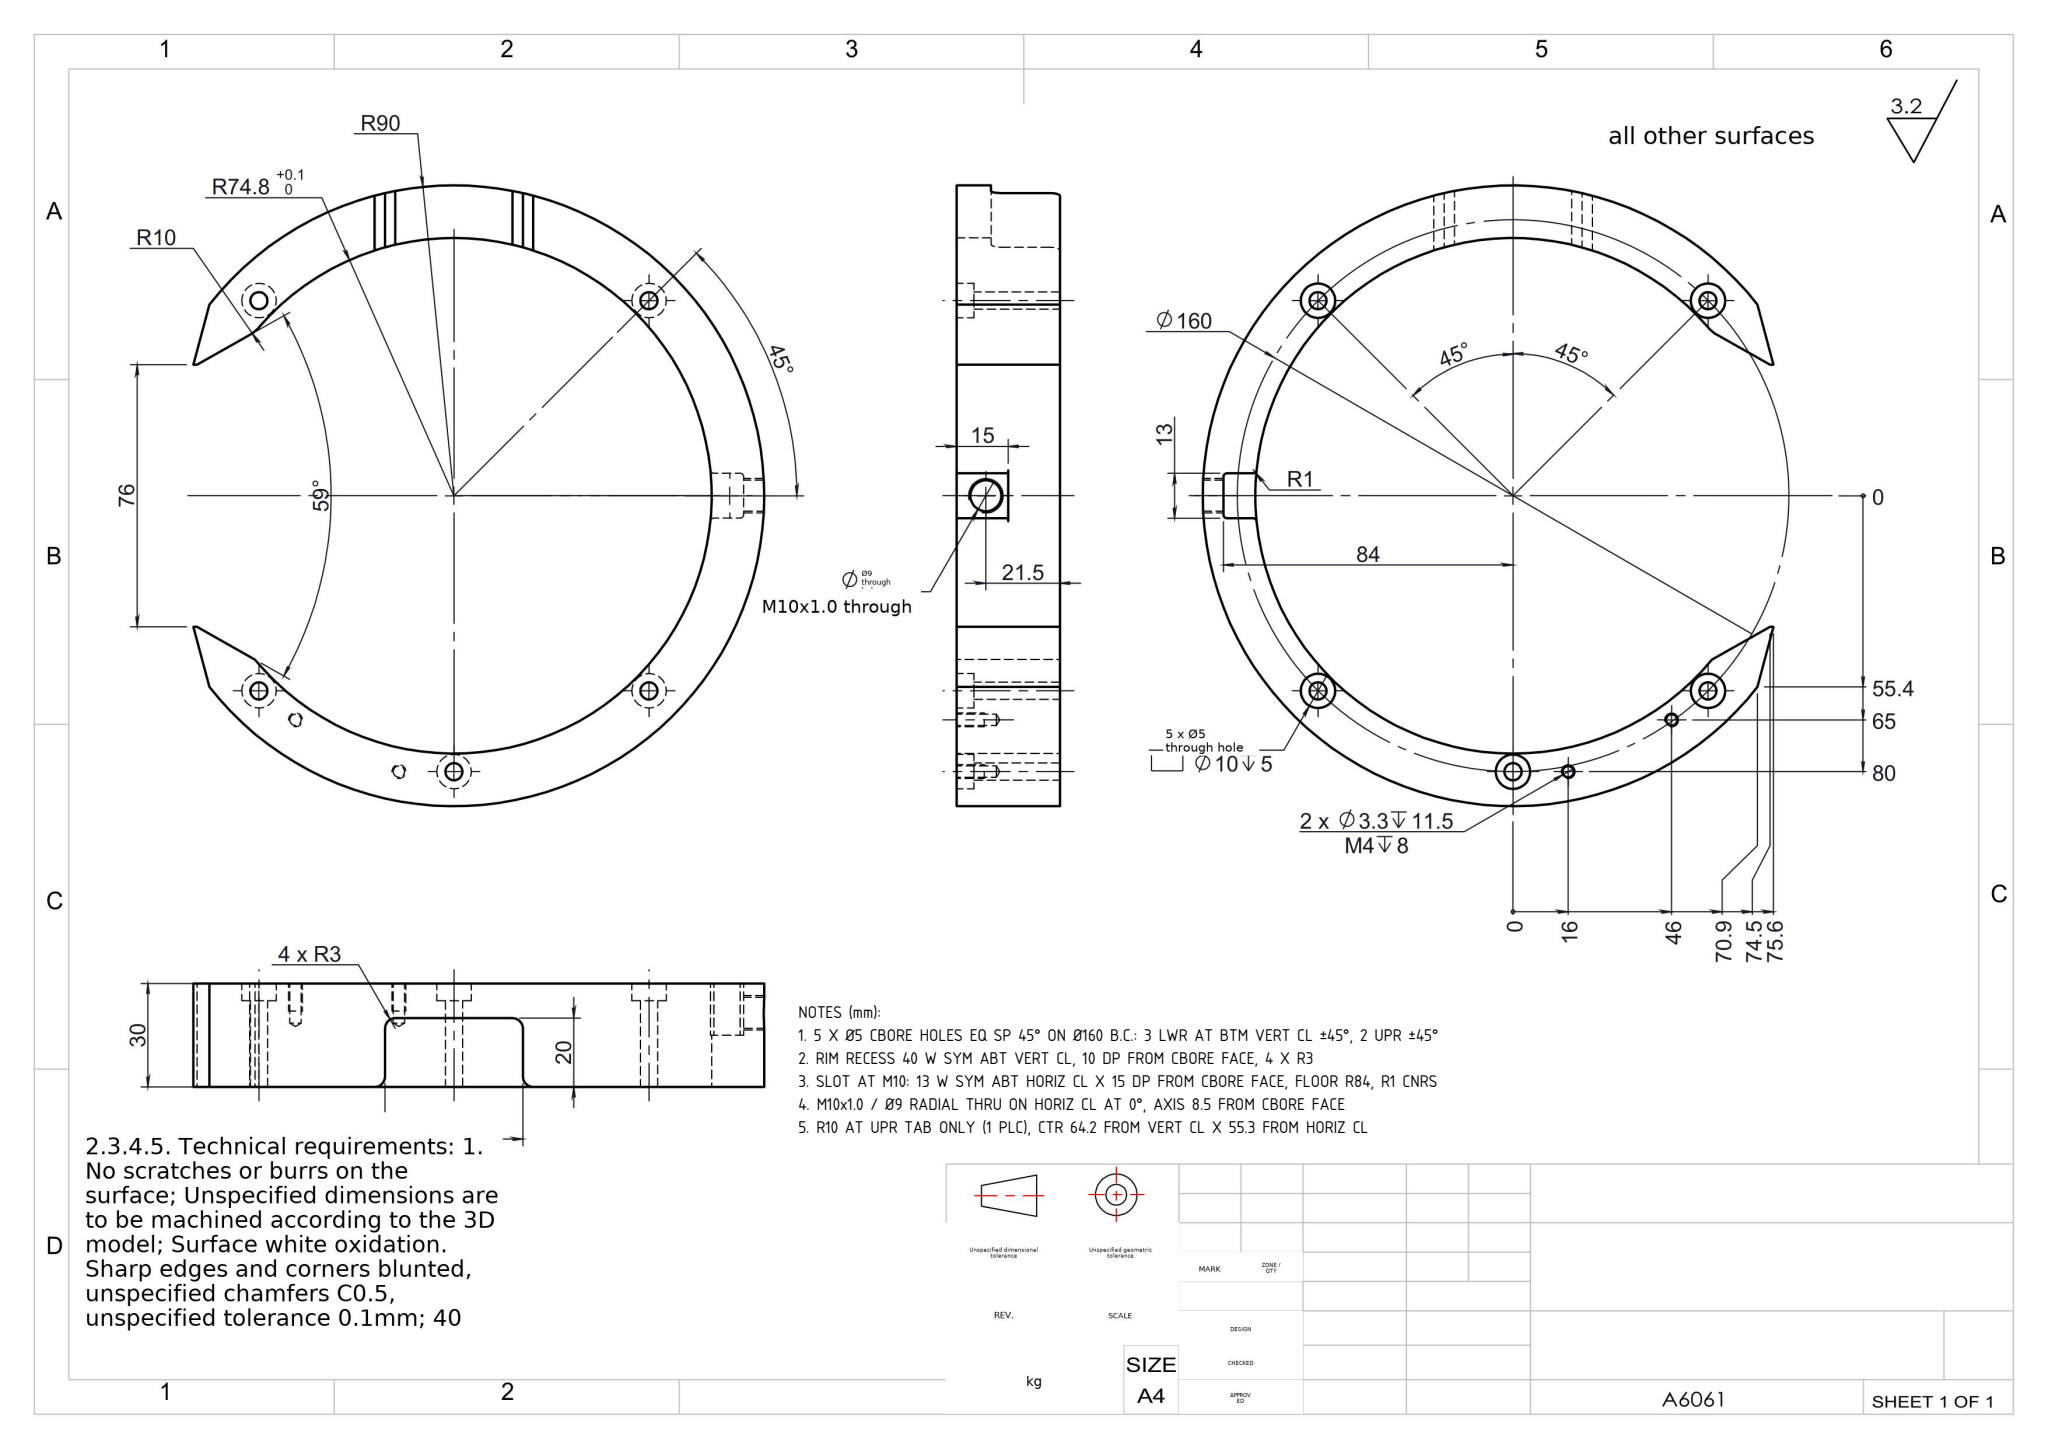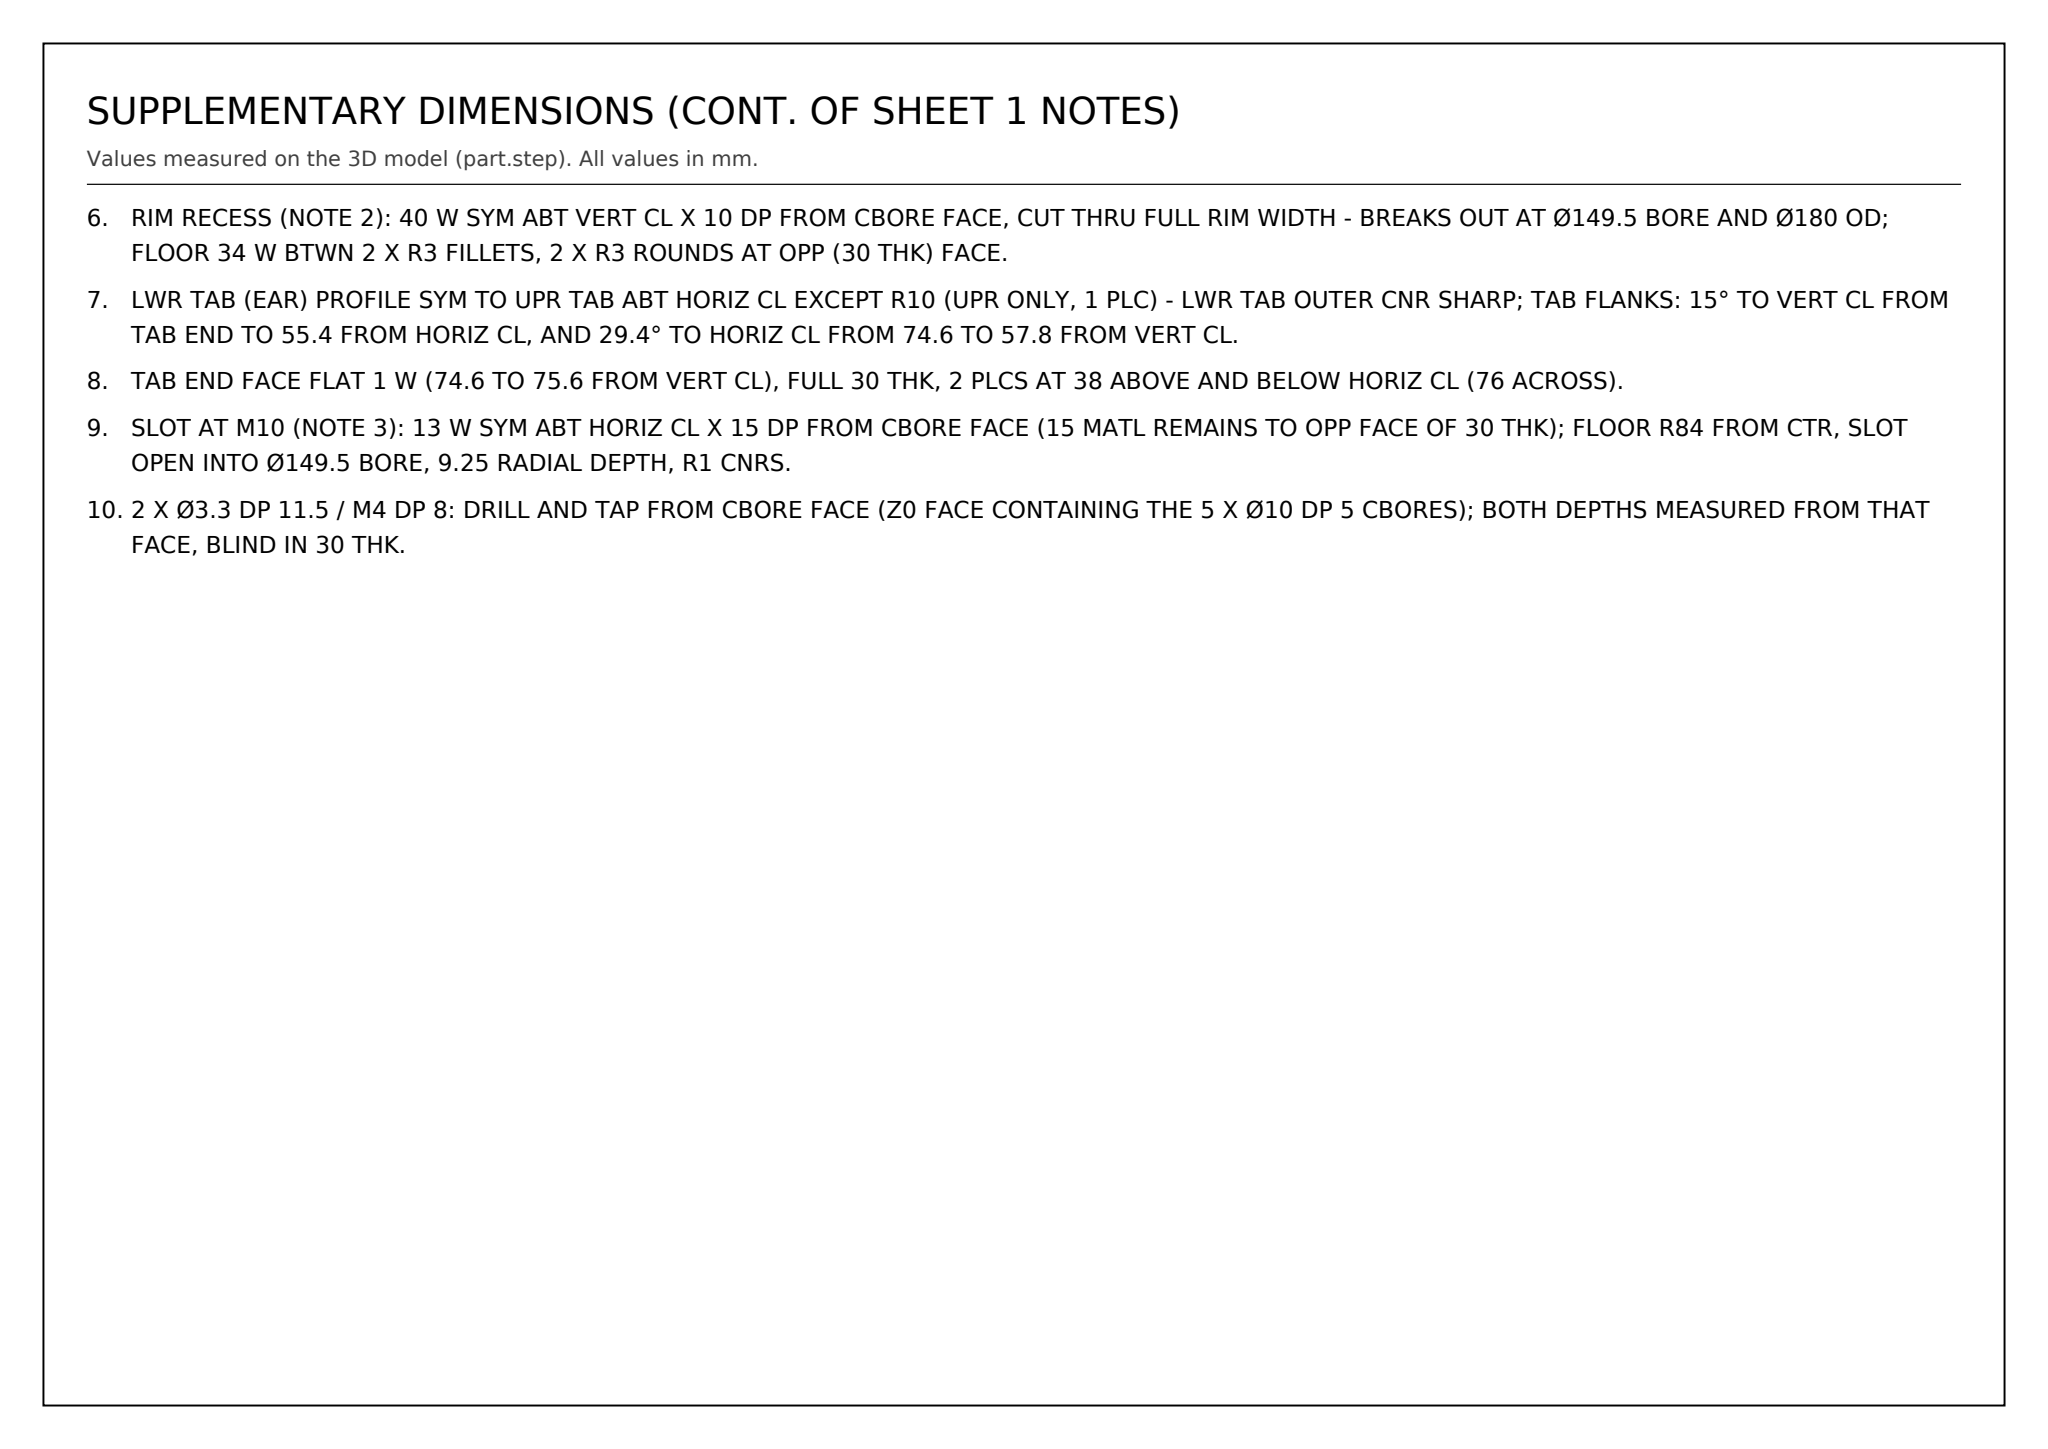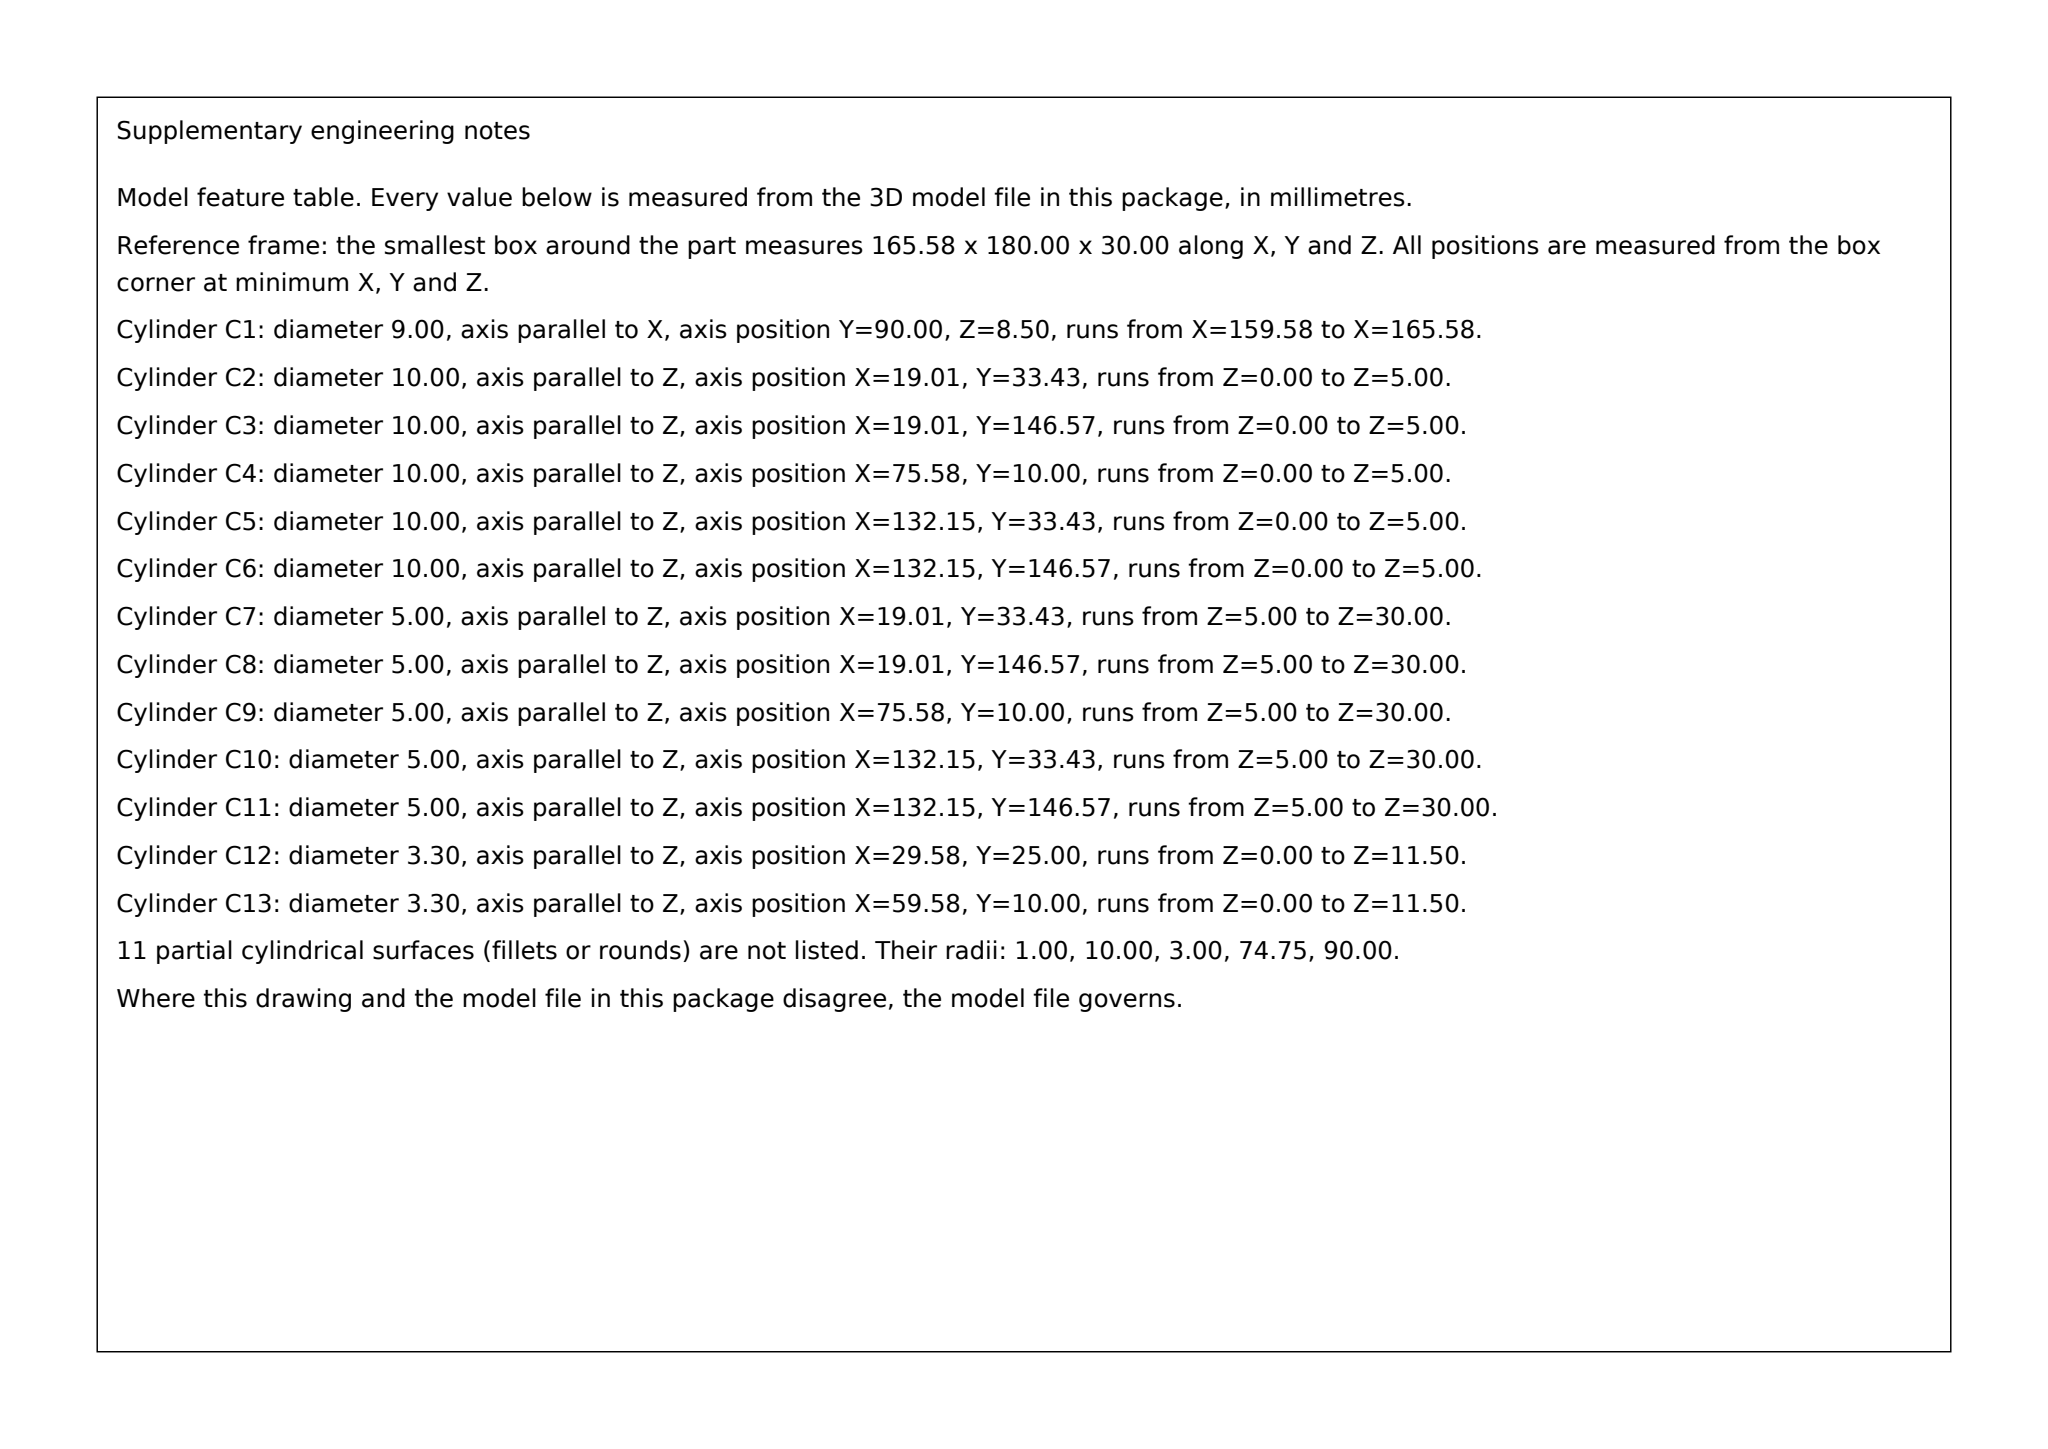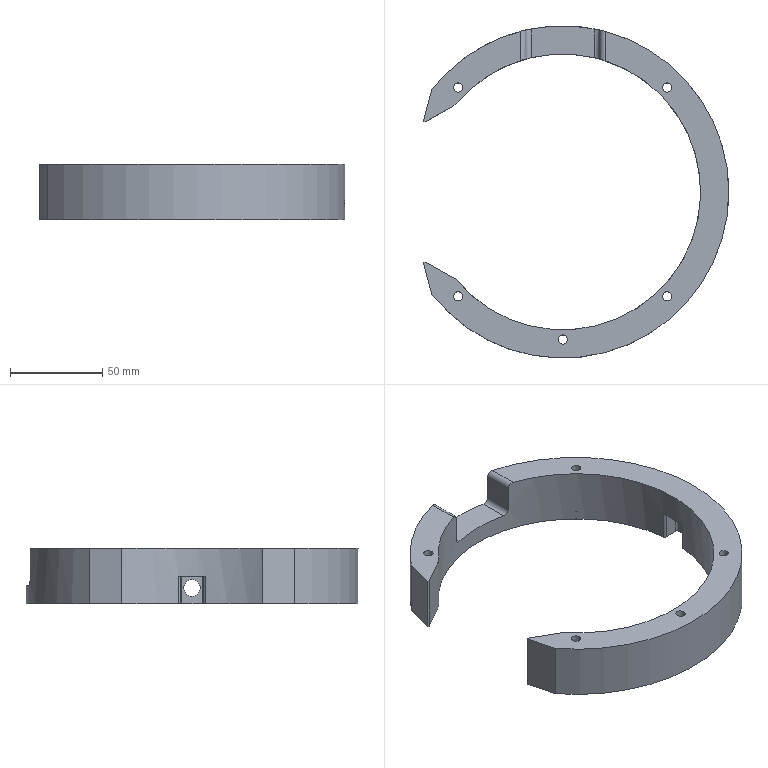Part | SolidWorks | mm | 1 solid | 62 faces | box 165.58 x 180 x 30 mm | volume 175087 mm3 | cylinder 37 | plane 21 | cone 4 | commonest cylinder face diameters 10 x10 5 x10 3.3 x4 6 x4 2 x4 9 x2 180 x1 149.5 x1
Drawing notes:
5 X Ø5 CBORE HOLES EQ SP 45° ON Ø160 B.C.: 3 LWR AT BTM VERT CL ±45°, 2 UPR ±45° | from the solid: Hole angles from axis (75.58,90): 45,135,225,270,315°; radius 80 -> Ø160 B.C.
RIM RECESS 40 W SYM ABT VERT CL, 10 DP FROM CBORE FACE, 4 X R3 | from the solid: x-planes 55.58 & 95.58 (±20 from axis x=75.58); floor z=10, part 0-30, cbores ⌴5 from z=0
SLOT AT M10: 13 W SYM ABT HORIZ CL X 15 DP FROM CBORE FACE, FLOOR R84, R1 CNRS | from the solid: y-planes 83.5/96.5 (13 w about y=90); R1 corner cyls length 15 from z=0; x-plane 159.58 = R84
M10x1.0 / Ø9 RADIAL THRU ON HORIZ CL AT 0°, AXIS 8.5 FROM CBORE FACE | from the solid: Ø9 cyl axis along x at y=90 (bore axis y), z=8.5 (=30-21.5), thru rim OD Ø180 to R84 slot
R10 AT UPR TAB ONLY (1 PLC), CTR 64.2 FROM VERT CL X 55.3 FROM HORIZ CL | from the solid: single Ø20 z-cyl at (11.38,145.32) L30; rel axis (75.58,90) = (-64.20,+55.32); no 2nd Ø20
RIM RECESS (NOTE 2): 40 W SYM ABT VERT CL X 10 DP FROM CBORE FACE, CUT THRU FULL RIM WIDTH - BREAKS OUT AT Ø149.5 BORE AND Ø180 OD; FLOOR 34 W BTWN 2 X R3 FILLETS, 2 X R3 ROUNDS AT OPP (30 THK) FACE. | from the solid: axis_planes z=10 extent x[58.6,92.6] y[162.8,180.0]; axis_planes x=55.6 & x=95.6 extent y[162.0,177.7] z[13,27]; Ø6 y-axis concave arcs at z=13 and Ø6 y-axis convex arcs at z=27 (R3)
LWR TAB (EAR) PROFILE SYM TO UPR TAB ABT HORIZ CL EXCEPT R10 (UPR ONLY, 1 PLC) - LWR TAB OUTER CNR SHARP; TAB FLANKS: 15° TO VERT CL FROM TAB END TO 55.4 FROM HORIZ CL, AND 29.4° TO HORIZ CL FROM 74.6 TO 57.8 FROM VERT CL. | from the solid: inclined_planes [15,75,90] bbox_from [0,34.6,0] size [4.7,17.4,30] (mirror [0,128,0]); inclined_planes [60.6,29.4,90] bbox_from [1,42.5,0] size [16.8,9.5,30] (upr [1,128,0] size [15.3,8.6,30]); convex arc Ø20 at (11.4,145.3) = R10 upr only
TAB END FACE FLAT 1 W (74.6 TO 75.6 FROM VERT CL), FULL 30 THK, 2 PLCS AT 38 ABOVE AND BELOW HORIZ CL (76 ACROSS). | from the solid: axis_planes y=52.0 and y=128.0, extent x[0.0,1.0] z[0.0,30.0]
SLOT AT M10 (NOTE 3): 13 W SYM ABT HORIZ CL X 15 DP FROM CBORE FACE (15 MATL REMAINS TO OPP FACE OF 30 THK); FLOOR R84 FROM CTR, SLOT OPEN INTO Ø149.5 BORE, 9.25 RADIAL DEPTH, R1 CNRS. | from the solid: axis_planes x=159.6 extent y[84.5,95.5] z[0,15] (R84 floor); axis_planes y=83.5 & y=96.5 extent x[151.0,158.6] z[0,15]; axis_planes z=15 extent x[150.0,159.6] y[82.6,97.4]; Ø2 z-axis arcs at (158.6,84.5)/(158.6,95.5) and (151.0,82.5)/(151.0,97.5)
2 X Ø3.3 DP 11.5 / M4 DP 8: DRILL AND TAP FROM CBORE FACE (Z0 FACE CONTAINING THE 5 X Ø10 DP 5 CBORES); BOTH DEPTHS MEASURED FROM THAT FACE, BLIND IN 30 THK. | from the solid: cylinders: hole/bore Ø3.3 axis z from 0.0 to 11.5 at (29.6,25.0) and (59.6,10.0); hole/bore Ø10 axis z from 0.0 to 5.0 (5 plcs) — same z=0 entry face; plane z=30 is opposite face